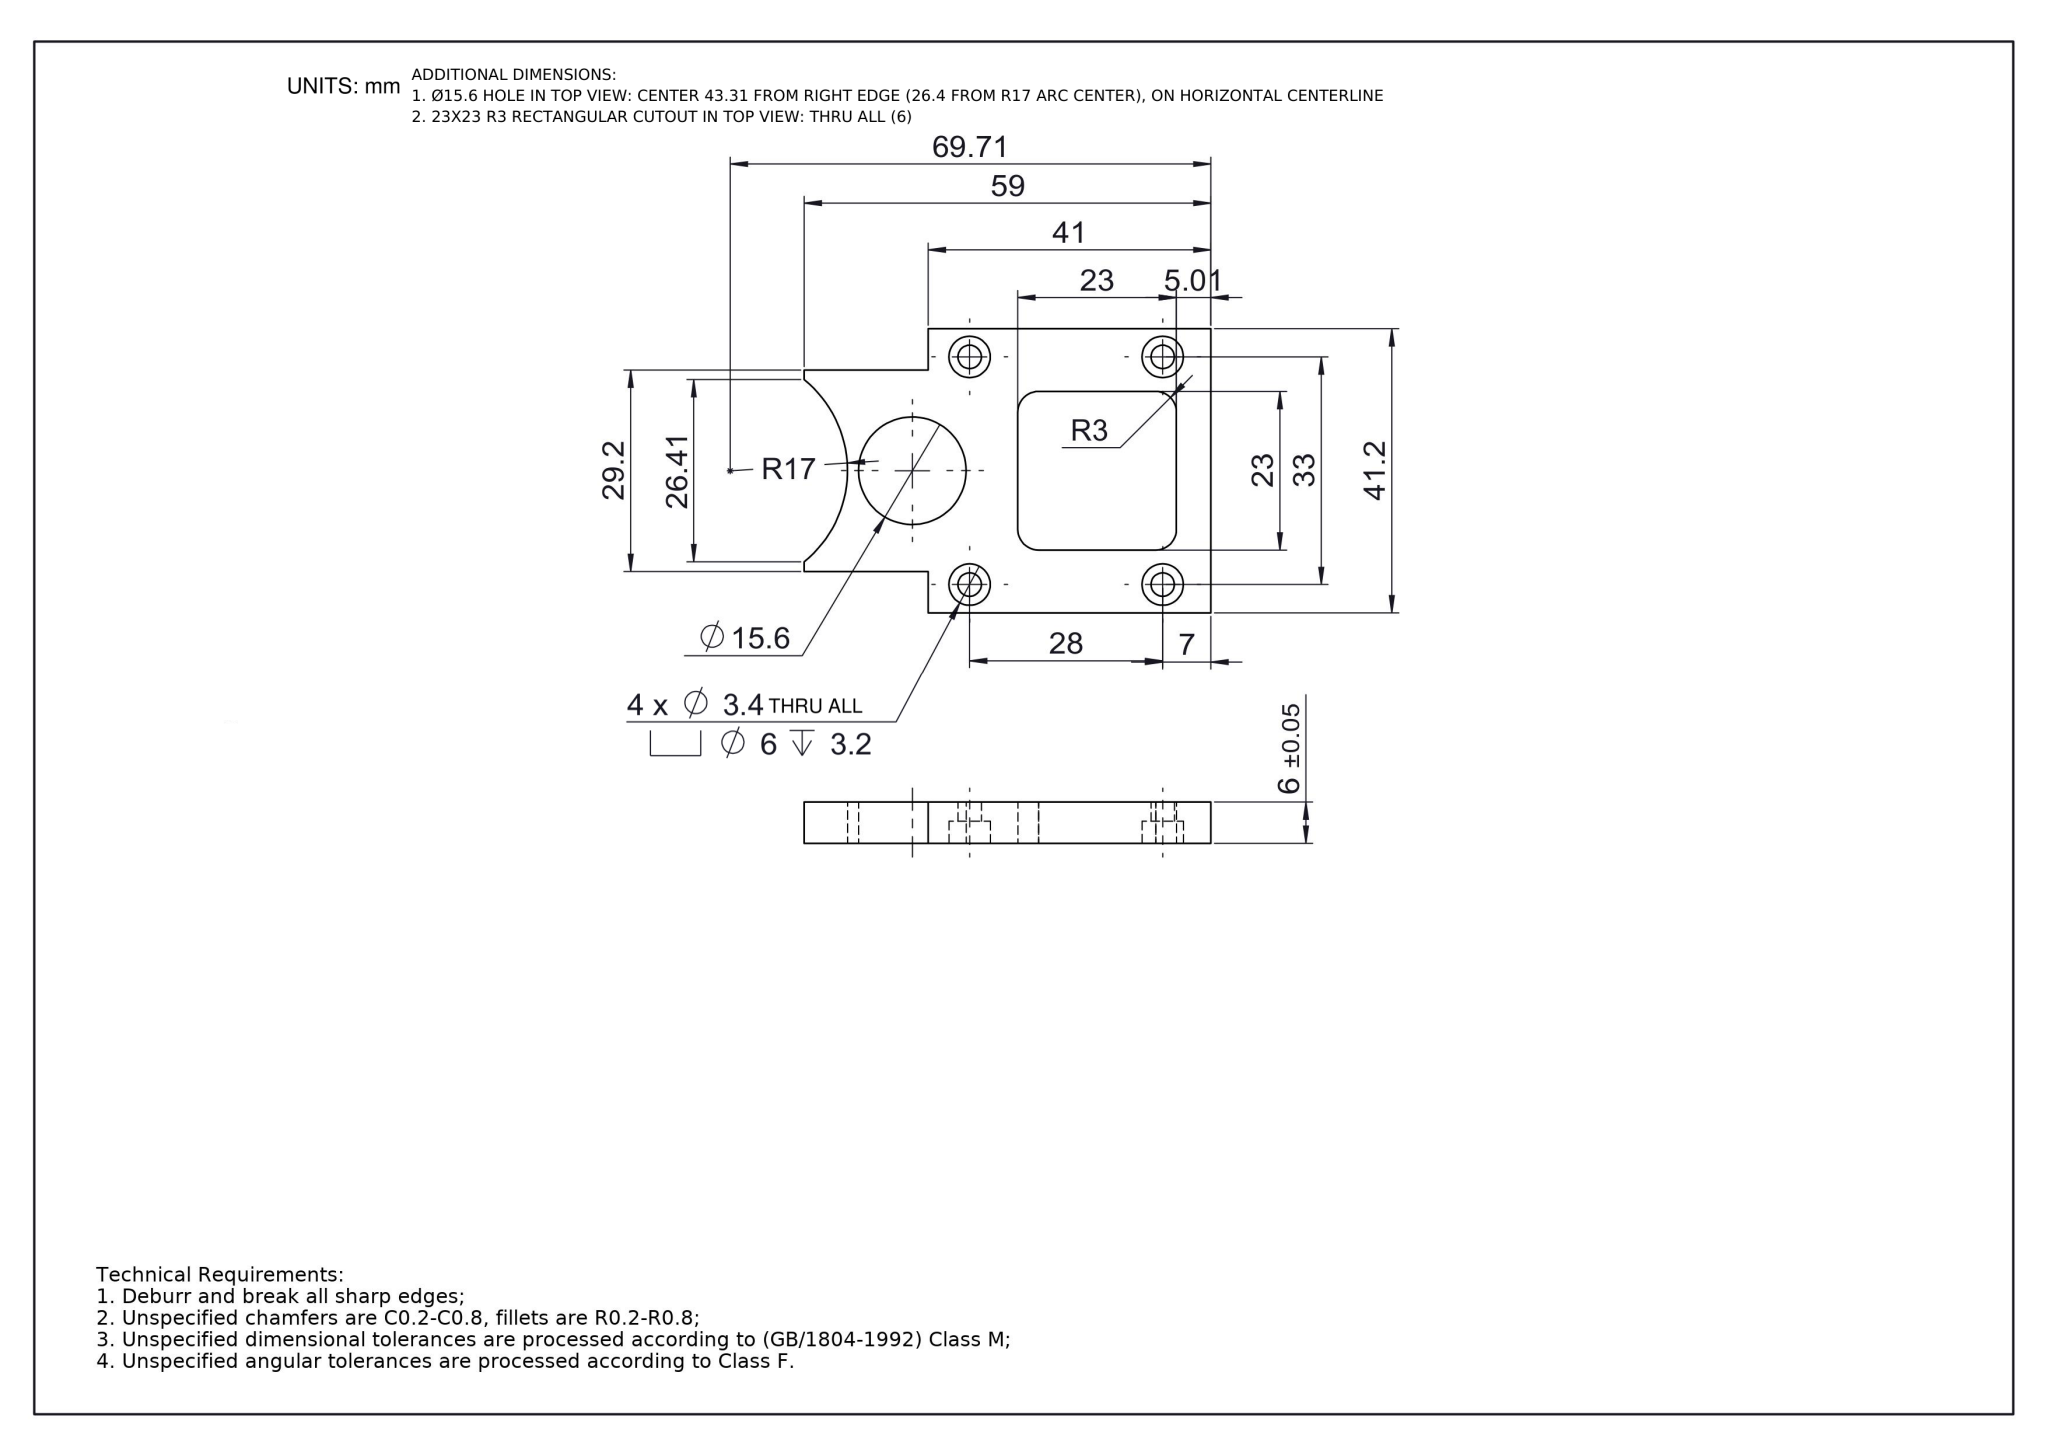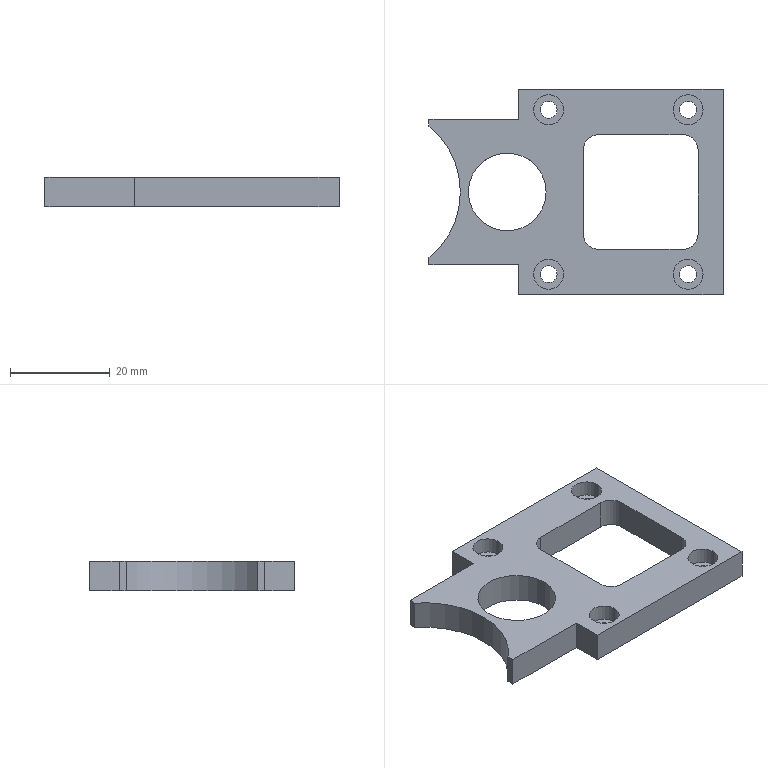Part | NX | mm | 1 solid | 42 faces | box 59 x 41.2 x 6 mm | volume 7857 mm3 | cylinder 23 | plane 19 | commonest cylinder face diameters 6 x12 3.4 x8 15.6 x2 34 x1